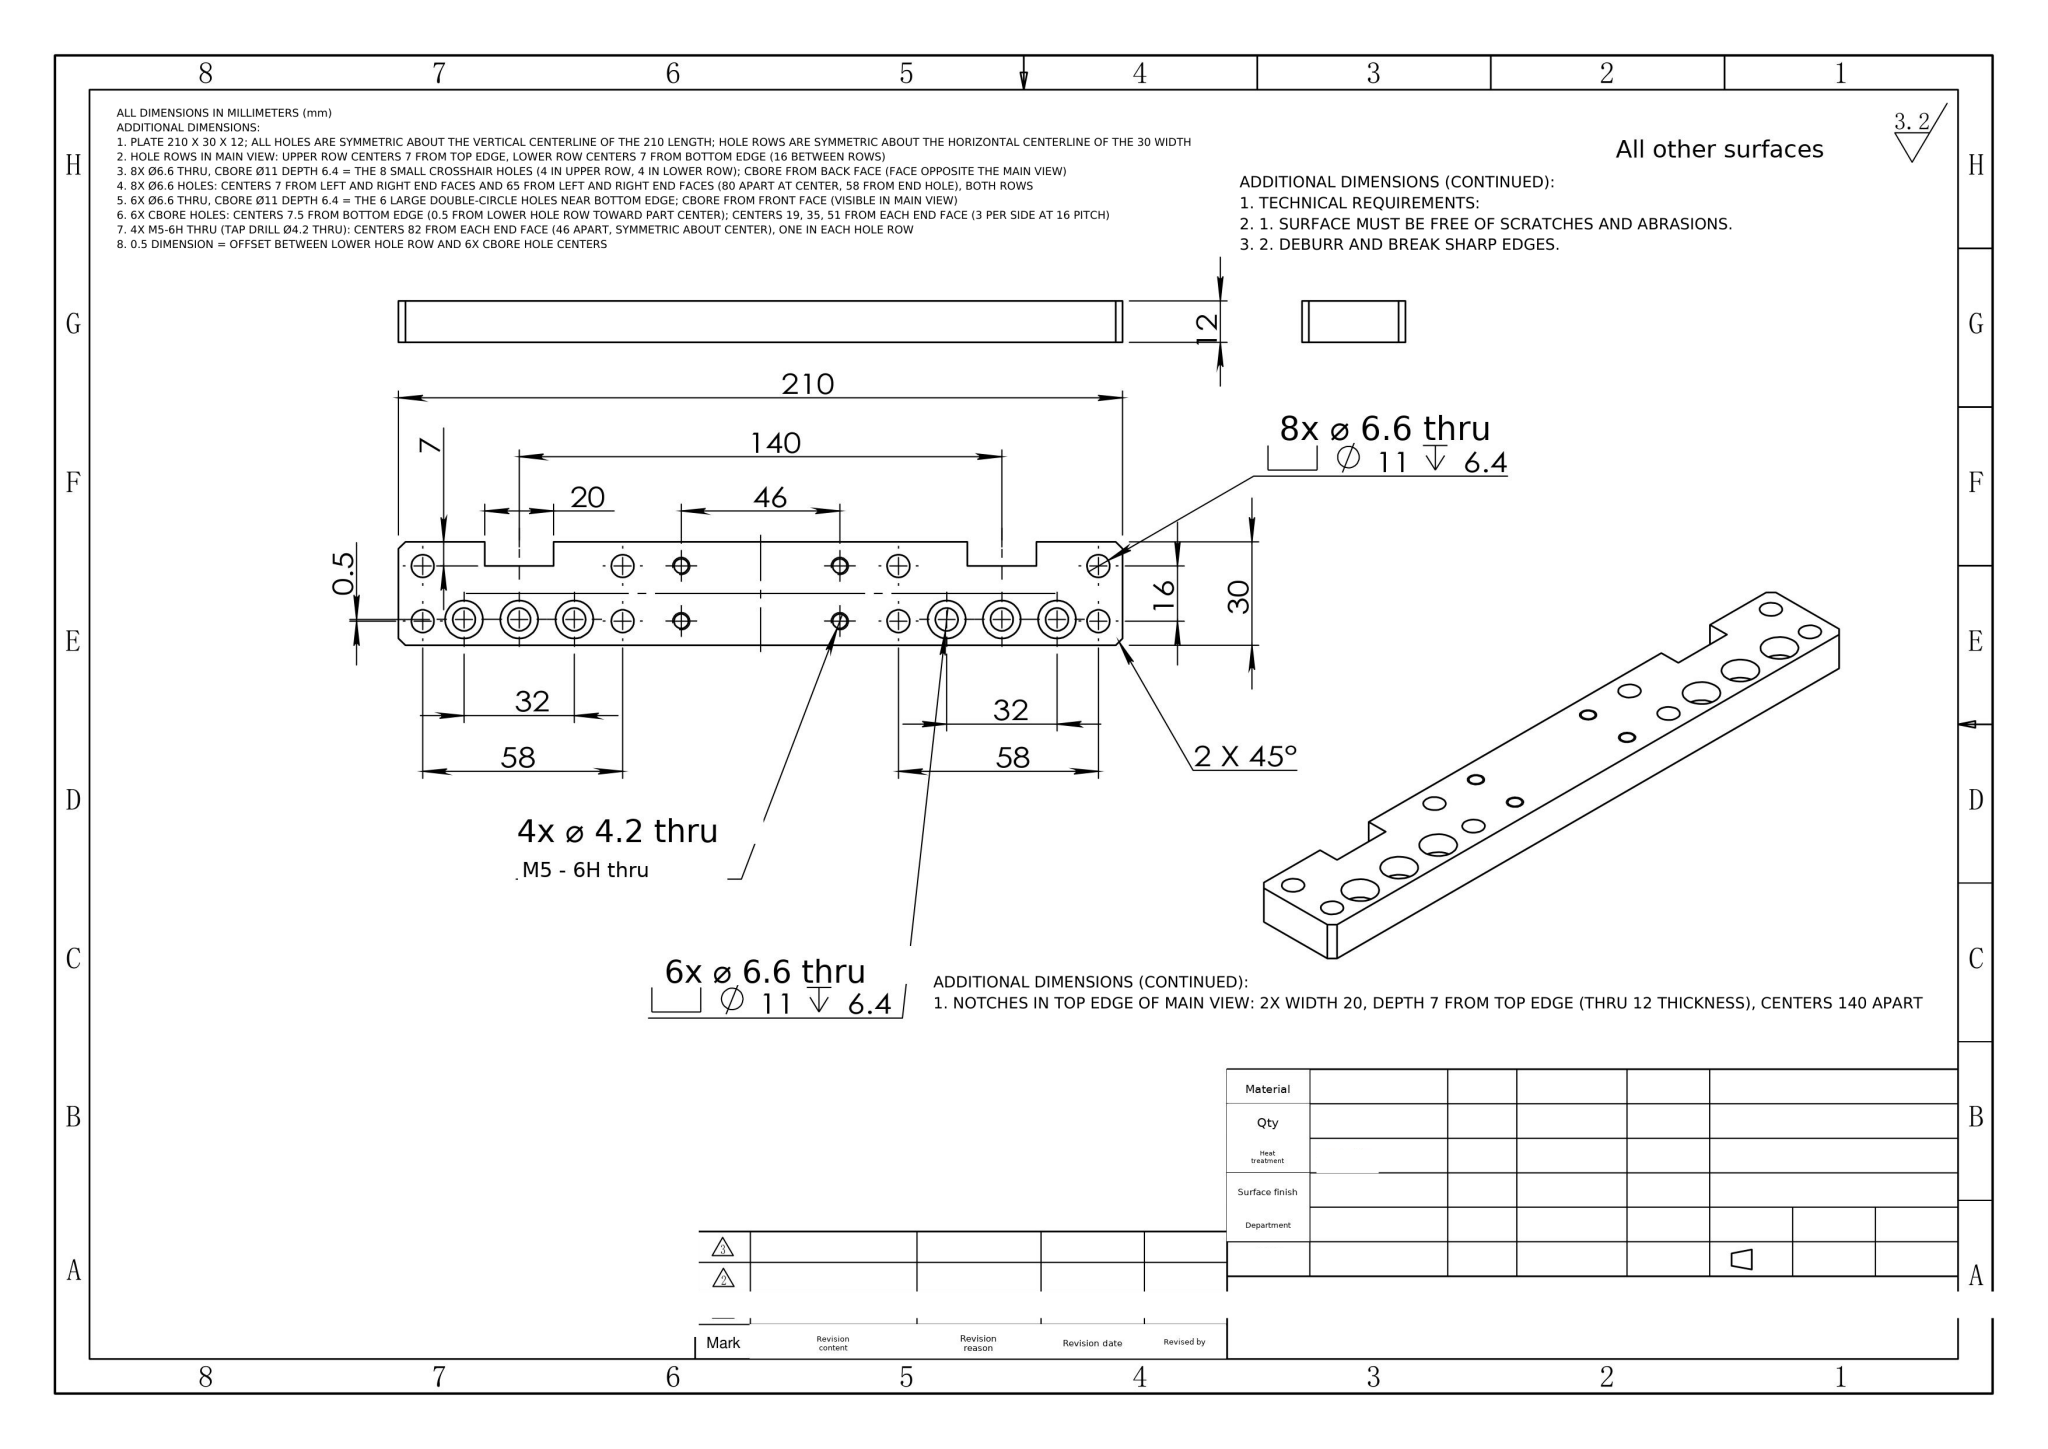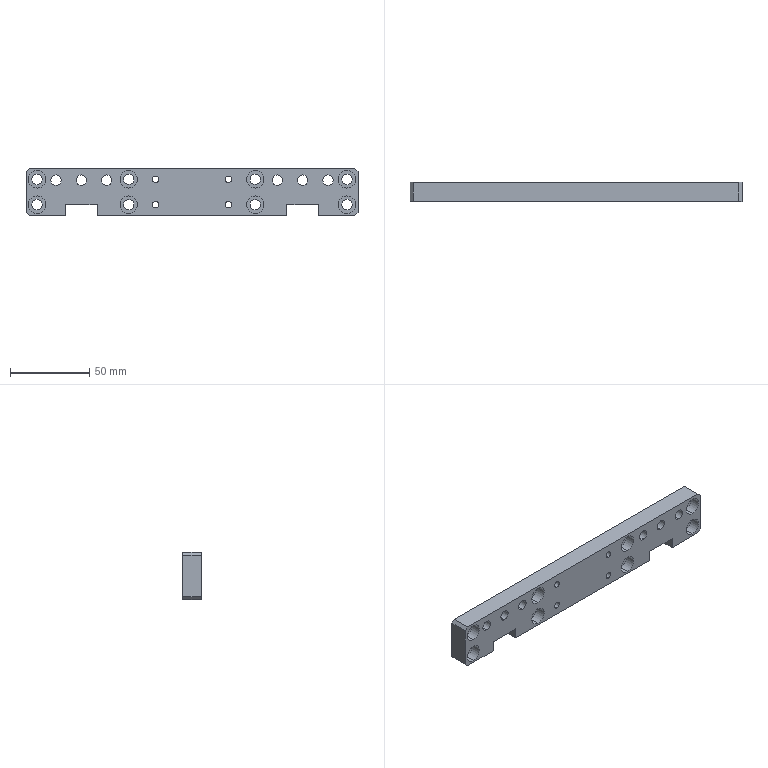Part | NX | mm | 1 solid | 96 faces | box 210 x 12 x 30 mm | volume 60282 mm3 | cylinder 64 | plane 32 | commonest cylinder face diameters 11 x28 6.6 x28 4.2 x8